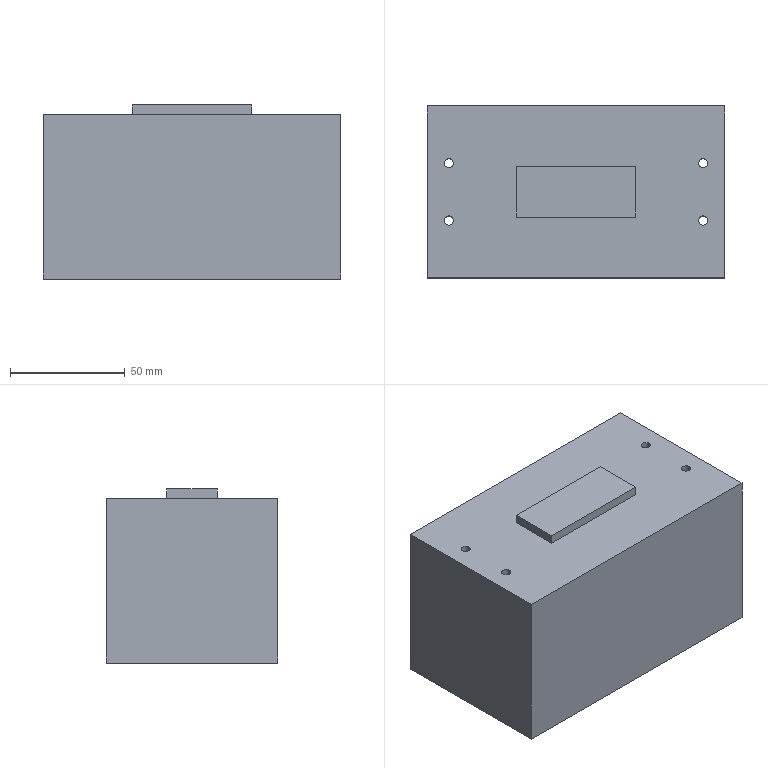Component | SolidWorks | Switch-1 | 1 solid | 19 faces | box 130 x 75 x 76 mm | volume 702957 mm3 | plane 11 | cylinder 8 | commonest cylinder face diameters 4 x8
build123d program:
from build123d import *

# Parameters (mm, degrees)
SKETCH1_W                 = 130
SKETCH1_H                 = 75
BOSS_EXTRUDE1_DEPTH       = 72
SKETCH2_W                 = 52
SKETCH2_H                 = 22
BOSS_EXTRUDE2_DEPTH       = 4
SKETCH3_R                 = 2
CUT_EXTRUDE1_DEPTH        = 80
LPATTERN1_COUNT           = 2
LPATTERN1_PITCH           = 25
LPATTERN2_COUNT           = 2
LPATTERN2_PITCH           = 111
LPATTERN2_COPY_1_SKETCH_R = 2
LPATTERN2_COPY_1_DEPTH    = 80


with BuildPart() as part:
    # Sketch1 → Boss-Extrude1 (new body)
    with BuildSketch(Plane.XY):
        Rectangle(SKETCH1_W, SKETCH1_H)
    extrude(amount=BOSS_EXTRUDE1_DEPTH)

    # Sketch2 → Boss-Extrude2 (add)
    with BuildSketch(Plane.XY.offset(72)):
        Rectangle(SKETCH2_W, SKETCH2_H)
    extrude(amount=BOSS_EXTRUDE2_DEPTH)

    # Sketch3 → Cut-Extrude1 (cut)
    with BuildSketch(Plane(origin=(0, 0, 0), x_dir=(-1, 0, 0), z_dir=(0, 0, -1))):
        with Locations((-55.5, -12.5)):
            Circle(SKETCH3_R)
    cut_extrude1 = extrude(amount=-CUT_EXTRUDE1_DEPTH, mode=Mode.SUBTRACT)

    # LPattern1: Cut-Extrude1 ×2
    with Locations(*[(0, i * LPATTERN1_PITCH, 0) for i in range(1, LPATTERN1_COUNT)]):
        add(cut_extrude1, mode=Mode.SUBTRACT)

    # LPattern2: Cut-Extrude1 ×2
    with Locations(*[(-i * LPATTERN2_PITCH, 0, 0) for i in range(1, LPATTERN2_COUNT)]):
        add(cut_extrude1, mode=Mode.SUBTRACT)

    # LPattern2 copy 1 sketch → LPattern2 copy 1 (cut)
    with BuildSketch(Plane(origin=(-111, 25, 0), x_dir=(-1, 0, 0), z_dir=(0, 0, -1))):
        with Locations((-55.5, -12.5)):
            Circle(LPATTERN2_COPY_1_SKETCH_R)
    extrude(amount=-LPATTERN2_COPY_1_DEPTH, mode=Mode.SUBTRACT)


solid = part.part

# Placed as in the assembly
solid = solid.moved(Location((172.727, 924.814, -141.5), (0, 0, 0)))
STEP:
#1=COLOUR_RGB('',0.7922,0.8196,0.9333);
#2=FILL_AREA_STYLE_COLOUR('',#1);
#3=FILL_AREA_STYLE('',(#2));
#4=SURFACE_STYLE_FILL_AREA(#3);
#5=SURFACE_SIDE_STYLE('',(#4));
#6=SURFACE_STYLE_USAGE(.BOTH.,#5);
#7=PRESENTATION_STYLE_ASSIGNMENT((#6));
#8=CARTESIAN_POINT('',(4.536,36.902,-2.736));
#9=VERTEX_POINT('',#8);
#10=CARTESIAN_POINT('',(4.694,36.902,-2.736));
#11=VERTEX_POINT('',#10);
#12=CARTESIAN_POINT('',(4.615,36.902,-2.736));
#13=DIRECTION('',(0.,0.,1.));
#14=DIRECTION('',(1.,0.,0.));
#15=AXIS2_PLACEMENT_3D('',#12,#13,#14);
#16=CIRCLE('',#15,0.07874);
#17=EDGE_CURVE('',#9,#11,#16,.T.);
#18=ORIENTED_EDGE('',*,*,#17,.T.);
#19=CARTESIAN_POINT('',(4.694,36.902,-5.571));
#20=VERTEX_POINT('',#19);
#21=CARTESIAN_POINT('',(4.694,36.902,-2.421));
#22=DIRECTION('',(0.,0.,-1.));
#23=VECTOR('',#22,39.37);
#24=LINE('',#21,#23);
#25=EDGE_CURVE('',#11,#20,#24,.T.);
#26=ORIENTED_EDGE('',*,*,#25,.T.);
#27=CARTESIAN_POINT('',(4.536,36.902,-5.571));
#28=VERTEX_POINT('',#27);
#29=CARTESIAN_POINT('',(4.615,36.902,-5.571));
#30=DIRECTION('',(0.,0.,-1.));
#31=DIRECTION('',(-1.,0.,0.));
#32=AXIS2_PLACEMENT_3D('',#29,#30,#31);
#33=CIRCLE('',#32,0.07874);
#34=EDGE_CURVE('',#20,#28,#33,.T.);
#35=ORIENTED_EDGE('',*,*,#34,.T.);
#36=CARTESIAN_POINT('',(4.536,36.902,-2.421));
#37=DIRECTION('',(0.,0.,-1.));
#38=VECTOR('',#37,39.37);
#39=LINE('',#36,#38);
#40=EDGE_CURVE('',#9,#28,#39,.T.);
#41=ORIENTED_EDGE('',*,*,#40,.F.);
#42=EDGE_LOOP('',(#18,#26,#35,#41));
#43=FACE_OUTER_BOUND('',#42,.T.);
#44=CARTESIAN_POINT('',(4.615,36.902,-2.421));
#45=DIRECTION('',(0.,0.,-1.));
#46=DIRECTION('',(-1.,0.,0.));
#47=AXIS2_PLACEMENT_3D('',#44,#45,#46);
#48=CYLINDRICAL_SURFACE('',#47,0.07874);
#49=ADVANCED_FACE('',(#43),#48,.F.);
#50=CARTESIAN_POINT('',(4.536,35.918,-2.736));
#51=VERTEX_POINT('',#50);
#52=CARTESIAN_POINT('',(4.694,35.918,-2.736));
#53=VERTEX_POINT('',#52);
#54=CARTESIAN_POINT('',(4.615,35.918,-2.736));
#55=DIRECTION('',(0.,0.,1.));
#56=DIRECTION('',(1.,0.,0.));
#57=AXIS2_PLACEMENT_3D('',#54,#55,#56);
#58=CIRCLE('',#57,0.07874);
#59=EDGE_CURVE('',#51,#53,#58,.T.);
#60=ORIENTED_EDGE('',*,*,#59,.T.);
#61=CARTESIAN_POINT('',(4.694,35.918,-5.571));
#62=VERTEX_POINT('',#61);
#63=CARTESIAN_POINT('',(4.694,35.918,-2.421));
#64=DIRECTION('',(0.,0.,-1.));
#65=VECTOR('',#64,39.37);
#66=LINE('',#63,#65);
#67=EDGE_CURVE('',#53,#62,#66,.T.);
#68=ORIENTED_EDGE('',*,*,#67,.T.);
#69=CARTESIAN_POINT('',(4.536,35.918,-5.571));
#70=VERTEX_POINT('',#69);
#71=CARTESIAN_POINT('',(4.615,35.918,-5.571));
#72=DIRECTION('',(0.,0.,-1.));
#73=DIRECTION('',(-1.,0.,0.));
#74=AXIS2_PLACEMENT_3D('',#71,#72,#73);
#75=CIRCLE('',#74,0.07874);
#76=EDGE_CURVE('',#62,#70,#75,.T.);
#77=ORIENTED_EDGE('',*,*,#76,.T.);
#78=CARTESIAN_POINT('',(4.536,35.918,-2.421));
#79=DIRECTION('',(0.,0.,-1.));
#80=VECTOR('',#79,39.37);
#81=LINE('',#78,#80);
#82=EDGE_CURVE('',#51,#70,#81,.T.);
#83=ORIENTED_EDGE('',*,*,#82,.F.);
#84=EDGE_LOOP('',(#60,#68,#77,#83));
#85=FACE_OUTER_BOUND('',#84,.T.);
#86=CARTESIAN_POINT('',(4.615,35.918,-2.421));
#87=DIRECTION('',(0.,0.,-1.));
#88=DIRECTION('',(-1.,0.,0.));
#89=AXIS2_PLACEMENT_3D('',#86,#87,#88);
#90=CYLINDRICAL_SURFACE('',#89,0.07874);
#91=ADVANCED_FACE('',(#85),#90,.F.);
#92=CARTESIAN_POINT('',(8.907,36.902,-2.736));
#93=VERTEX_POINT('',#92);
#94=CARTESIAN_POINT('',(9.064,36.902,-2.736));
#95=VERTEX_POINT('',#94);
#96=CARTESIAN_POINT('',(8.985,36.902,-2.736));
#97=DIRECTION('',(0.,0.,1.));
#98=DIRECTION('',(1.,0.,0.));
#99=AXIS2_PLACEMENT_3D('',#96,#97,#98);
#100=CIRCLE('',#99,0.07874);
#101=EDGE_CURVE('',#93,#95,#100,.T.);
#102=ORIENTED_EDGE('',*,*,#101,.T.);
#103=CARTESIAN_POINT('',(9.064,36.902,-5.571));
#104=VERTEX_POINT('',#103);
#105=CARTESIAN_POINT('',(9.064,36.902,-2.421));
#106=DIRECTION('',(0.,0.,-1.));
#107=VECTOR('',#106,39.37);
#108=LINE('',#105,#107);
#109=EDGE_CURVE('',#95,#104,#108,.T.);
#110=ORIENTED_EDGE('',*,*,#109,.T.);
#111=CARTESIAN_POINT('',(8.907,36.902,-5.571));
#112=VERTEX_POINT('',#111);
#113=CARTESIAN_POINT('',(8.985,36.902,-5.571));
#114=DIRECTION('',(0.,0.,-1.));
#115=DIRECTION('',(-1.,0.,0.));
#116=AXIS2_PLACEMENT_3D('',#113,#114,#115);
#117=CIRCLE('',#116,0.07874);
#118=EDGE_CURVE('',#104,#112,#117,.T.);
#119=ORIENTED_EDGE('',*,*,#118,.T.);
#120=CARTESIAN_POINT('',(8.907,36.902,-2.421));
#121=DIRECTION('',(0.,0.,-1.));
#122=VECTOR('',#121,39.37);
#123=LINE('',#120,#122);
#124=EDGE_CURVE('',#93,#112,#123,.T.);
#125=ORIENTED_EDGE('',*,*,#124,.F.);
#126=EDGE_LOOP('',(#102,#110,#119,#125));
#127=FACE_OUTER_BOUND('',#126,.T.);
#128=CARTESIAN_POINT('',(8.985,36.902,-2.421));
#129=DIRECTION('',(0.,0.,-1.));
#130=DIRECTION('',(-1.,0.,0.));
#131=AXIS2_PLACEMENT_3D('',#128,#129,#130);
#132=CYLINDRICAL_SURFACE('',#131,0.07874);
#133=ADVANCED_FACE('',(#127),#132,.F.);
#134=CARTESIAN_POINT('',(8.907,35.918,-2.736));
#135=VERTEX_POINT('',#134);
#136=CARTESIAN_POINT('',(9.064,35.918,-2.736));
#137=VERTEX_POINT('',#136);
#138=CARTESIAN_POINT('',(8.985,35.918,-2.736));
#139=DIRECTION('',(0.,0.,1.));
#140=DIRECTION('',(1.,0.,0.));
#141=AXIS2_PLACEMENT_3D('',#138,#139,#140);
#142=CIRCLE('',#141,0.07874);
#143=EDGE_CURVE('',#135,#137,#142,.T.);
#144=ORIENTED_EDGE('',*,*,#143,.T.);
#145=CARTESIAN_POINT('',(9.064,35.918,-5.571));
#146=VERTEX_POINT('',#145);
#147=CARTESIAN_POINT('',(9.064,35.918,-2.421));
#148=DIRECTION('',(0.,0.,-1.));
#149=VECTOR('',#148,39.37);
#150=LINE('',#147,#149);
#151=EDGE_CURVE('',#137,#146,#150,.T.);
#152=ORIENTED_EDGE('',*,*,#151,.T.);
#153=CARTESIAN_POINT('',(8.907,35.918,-5.571));
#154=VERTEX_POINT('',#153);
#155=CARTESIAN_POINT('',(8.985,35.918,-5.571));
#156=DIRECTION('',(0.,0.,-1.));
#157=DIRECTION('',(-1.,0.,0.));
#158=AXIS2_PLACEMENT_3D('',#155,#156,#157);
#159=CIRCLE('',#158,0.07874);
#160=EDGE_CURVE('',#146,#154,#159,.T.);
#161=ORIENTED_EDGE('',*,*,#160,.T.);
#162=CARTESIAN_POINT('',(8.907,35.918,-2.421));
#163=DIRECTION('',(0.,0.,-1.));
#164=VECTOR('',#163,39.37);
#165=LINE('',#162,#164);
#166=EDGE_CURVE('',#135,#154,#165,.T.);
#167=ORIENTED_EDGE('',*,*,#166,.F.);
#168=EDGE_LOOP('',(#144,#152,#161,#167));
#169=FACE_OUTER_BOUND('',#168,.T.);
#170=CARTESIAN_POINT('',(8.985,35.918,-2.421));
#171=DIRECTION('',(0.,0.,-1.));
#172=DIRECTION('',(-1.,0.,0.));
#173=AXIS2_PLACEMENT_3D('',#170,#171,#172);
#174=CYLINDRICAL_SURFACE('',#173,0.07874);
#175=ADVANCED_FACE('',(#169),#174,.F.);
#176=ORIENTED_EDGE('',*,*,#17,.F.);
#177=CARTESIAN_POINT('',(4.615,36.902,-2.736));
#178=DIRECTION('',(0.,0.,1.));
#179=DIRECTION('',(1.,0.,0.));
#180=AXIS2_PLACEMENT_3D('',#177,#178,#179);
#181=CIRCLE('',#180,0.07874);
#182=EDGE_CURVE('',#11,#9,#181,.T.);
#183=ORIENTED_EDGE('',*,*,#182,.F.);
#184=EDGE_LOOP('',(#176,#183));
#185=FACE_BOUND('',#184,.T.);
#186=ORIENTED_EDGE('',*,*,#59,.F.);
#187=CARTESIAN_POINT('',(4.615,35.918,-2.736));
#188=DIRECTION('',(0.,0.,1.));
#189=DIRECTION('',(1.,0.,0.));
#190=AXIS2_PLACEMENT_3D('',#187,#188,#189);
#191=CIRCLE('',#190,0.07874);
#192=EDGE_CURVE('',#53,#51,#191,.T.);
#193=ORIENTED_EDGE('',*,*,#192,.F.);
#194=EDGE_LOOP('',(#186,#193));
#195=FACE_BOUND('',#194,.T.);
#196=ORIENTED_EDGE('',*,*,#101,.F.);
#197=CARTESIAN_POINT('',(8.985,36.902,-2.736));
#198=DIRECTION('',(0.,0.,1.));
#199=DIRECTION('',(1.,0.,0.));
#200=AXIS2_PLACEMENT_3D('',#197,#198,#199);
#201=CIRCLE('',#200,0.07874);
#202=EDGE_CURVE('',#95,#93,#201,.T.);
#203=ORIENTED_EDGE('',*,*,#202,.F.);
#204=EDGE_LOOP('',(#196,#203));
#205=FACE_BOUND('',#204,.T.);
#206=ORIENTED_EDGE('',*,*,#143,.F.);
#207=CARTESIAN_POINT('',(8.985,35.918,-2.736));
#208=DIRECTION('',(0.,0.,1.));
#209=DIRECTION('',(1.,0.,0.));
#210=AXIS2_PLACEMENT_3D('',#207,#208,#209);
#211=CIRCLE('',#210,0.07874);
#212=EDGE_CURVE('',#137,#135,#211,.T.);
#213=ORIENTED_EDGE('',*,*,#212,.F.);
#214=EDGE_LOOP('',(#206,#213));
#215=FACE_BOUND('',#214,.T.);
#216=CARTESIAN_POINT('',(9.359,34.934,-2.736));
#217=VERTEX_POINT('',#216);
#218=CARTESIAN_POINT('',(9.359,37.886,-2.736));
#219=VERTEX_POINT('',#218);
#220=CARTESIAN_POINT('',(9.359,37.886,-2.736));
#221=DIRECTION('',(-0.,1.,0.));
#222=VECTOR('',#221,39.37);
#223=LINE('',#220,#222);
#224=EDGE_CURVE('',#217,#219,#223,.T.);
#225=ORIENTED_EDGE('',*,*,#224,.T.);
#226=CARTESIAN_POINT('',(4.241,37.886,-2.736));
#227=VERTEX_POINT('',#226);
#228=CARTESIAN_POINT('',(4.241,37.886,-2.736));
#229=DIRECTION('',(-1.,0.,0.));
#230=VECTOR('',#229,39.37);
#231=LINE('',#228,#230);
#232=EDGE_CURVE('',#219,#227,#231,.T.);
#233=ORIENTED_EDGE('',*,*,#232,.T.);
#234=CARTESIAN_POINT('',(4.241,34.934,-2.736));
#235=VERTEX_POINT('',#234);
#236=CARTESIAN_POINT('',(4.241,37.886,-2.736));
#237=DIRECTION('',(0.,-1.,0.));
#238=VECTOR('',#237,39.37);
#239=LINE('',#236,#238);
#240=EDGE_CURVE('',#227,#235,#239,.T.);
#241=ORIENTED_EDGE('',*,*,#240,.T.);
#242=CARTESIAN_POINT('',(4.241,34.934,-2.736));
#243=DIRECTION('',(1.,0.,0.));
#244=VECTOR('',#243,39.37);
#245=LINE('',#242,#244);
#246=EDGE_CURVE('',#235,#217,#245,.T.);
#247=ORIENTED_EDGE('',*,*,#246,.T.);
#248=EDGE_LOOP('',(#225,#233,#241,#247));
#249=FACE_OUTER_BOUND('',#248,.T.);
#250=CARTESIAN_POINT('',(7.824,36.843,-2.736));
#251=VERTEX_POINT('',#250);
#252=CARTESIAN_POINT('',(5.777,36.843,-2.736));
#253=VERTEX_POINT('',#252);
#254=CARTESIAN_POINT('',(5.777,36.843,-2.736));
#255=DIRECTION('',(-1.,0.,0.));
#256=VECTOR('',#255,39.37);
#257=LINE('',#254,#256);
#258=EDGE_CURVE('',#251,#253,#257,.T.);
#259=ORIENTED_EDGE('',*,*,#258,.F.);
#260=CARTESIAN_POINT('',(7.824,35.977,-2.736));
#261=VERTEX_POINT('',#260);
#262=CARTESIAN_POINT('',(7.824,36.843,-2.736));
#263=DIRECTION('',(0.,1.,0.));
#264=VECTOR('',#263,39.37);
#265=LINE('',#262,#264);
#266=EDGE_CURVE('',#261,#251,#265,.T.);
#267=ORIENTED_EDGE('',*,*,#266,.F.);
#268=CARTESIAN_POINT('',(5.777,35.977,-2.736));
#269=VERTEX_POINT('',#268);
#270=CARTESIAN_POINT('',(5.777,35.977,-2.736));
#271=DIRECTION('',(1.,0.,0.));
#272=VECTOR('',#271,39.37);
#273=LINE('',#270,#272);
#274=EDGE_CURVE('',#269,#261,#273,.T.);
#275=ORIENTED_EDGE('',*,*,#274,.F.);
#276=CARTESIAN_POINT('',(5.777,36.843,-2.736));
#277=DIRECTION('',(0.,-1.,0.));
#278=VECTOR('',#277,39.37);
#279=LINE('',#276,#278);
#280=EDGE_CURVE('',#253,#269,#279,.T.);
#281=ORIENTED_EDGE('',*,*,#280,.F.);
#282=EDGE_LOOP('',(#259,#267,#275,#281));
#283=FACE_BOUND('',#282,.T.);
#284=CARTESIAN_POINT('',(6.8,36.41,-2.736));
#285=DIRECTION('',(0.,0.,1.));
#286=DIRECTION('',(1.,0.,0.));
#287=AXIS2_PLACEMENT_3D('',#284,#285,#286);
#288=PLANE('',#287);
#289=ADVANCED_FACE('',(#185,#195,#205,#215,#249,#283),#288,.T.);
#290=CARTESIAN_POINT('',(9.359,34.934,-5.571));
#291=VERTEX_POINT('',#290);
#292=CARTESIAN_POINT('',(9.359,37.886,-5.571));
#293=VERTEX_POINT('',#292);
#294=CARTESIAN_POINT('',(9.359,37.886,-5.571));
#295=DIRECTION('',(-0.,1.,0.));
#296=VECTOR('',#295,39.37);
#297=LINE('',#294,#296);
#298=EDGE_CURVE('',#291,#293,#297,.T.);
#299=ORIENTED_EDGE('',*,*,#298,.T.);
#300=CARTESIAN_POINT('',(9.359,37.886,-2.736));
#301=DIRECTION('',(0.,0.,-1.));
#302=VECTOR('',#301,39.37);
#303=LINE('',#300,#302);
#304=EDGE_CURVE('',#219,#293,#303,.T.);
#305=ORIENTED_EDGE('',*,*,#304,.F.);
#306=ORIENTED_EDGE('',*,*,#224,.F.);
#307=CARTESIAN_POINT('',(9.359,34.934,-2.736));
#308=DIRECTION('',(0.,0.,-1.));
#309=VECTOR('',#308,39.37);
#310=LINE('',#307,#309);
#311=EDGE_CURVE('',#217,#291,#310,.T.);
#312=ORIENTED_EDGE('',*,*,#311,.T.);
#313=EDGE_LOOP('',(#299,#305,#306,#312));
#314=FACE_OUTER_BOUND('',#313,.T.);
#315=CARTESIAN_POINT('',(9.359,37.886,-2.736));
#316=DIRECTION('',(-1.,-0.,0.));
#317=DIRECTION('',(0.,-1.,0.));
#318=AXIS2_PLACEMENT_3D('',#315,#316,#317);
#319=PLANE('',#318);
#320=ADVANCED_FACE('',(#314),#319,.F.);
#321=CARTESIAN_POINT('',(4.241,37.886,-5.571));
#322=VERTEX_POINT('',#321);
#323=CARTESIAN_POINT('',(4.241,37.886,-5.571));
#324=DIRECTION('',(-1.,0.,0.));
#325=VECTOR('',#324,39.37);
#326=LINE('',#323,#325);
#327=EDGE_CURVE('',#293,#322,#326,.T.);
#328=ORIENTED_EDGE('',*,*,#327,.T.);
#329=CARTESIAN_POINT('',(4.241,37.886,-2.736));
#330=DIRECTION('',(0.,0.,-1.));
#331=VECTOR('',#330,39.37);
#332=LINE('',#329,#331);
#333=EDGE_CURVE('',#227,#322,#332,.T.);
#334=ORIENTED_EDGE('',*,*,#333,.F.);
#335=ORIENTED_EDGE('',*,*,#232,.F.);
#336=ORIENTED_EDGE('',*,*,#304,.T.);
#337=EDGE_LOOP('',(#328,#334,#335,#336));
#338=FACE_OUTER_BOUND('',#337,.T.);
#339=CARTESIAN_POINT('',(4.241,37.886,-2.736));
#340=DIRECTION('',(0.,-1.,0.));
#341=DIRECTION('',(0.,0.,-1.));
#342=AXIS2_PLACEMENT_3D('',#339,#340,#341);
#343=PLANE('',#342);
#344=ADVANCED_FACE('',(#338),#343,.F.);
#345=CARTESIAN_POINT('',(4.241,34.934,-5.571));
#346=VERTEX_POINT('',#345);
#347=CARTESIAN_POINT('',(4.241,37.886,-5.571));
#348=DIRECTION('',(0.,-1.,0.));
#349=VECTOR('',#348,39.37);
#350=LINE('',#347,#349);
#351=EDGE_CURVE('',#322,#346,#350,.T.);
#352=ORIENTED_EDGE('',*,*,#351,.T.);
#353=CARTESIAN_POINT('',(4.241,34.934,-2.736));
#354=DIRECTION('',(0.,0.,-1.));
#355=VECTOR('',#354,39.37);
#356=LINE('',#353,#355);
#357=EDGE_CURVE('',#235,#346,#356,.T.);
#358=ORIENTED_EDGE('',*,*,#357,.F.);
#359=ORIENTED_EDGE('',*,*,#240,.F.);
#360=ORIENTED_EDGE('',*,*,#333,.T.);
#361=EDGE_LOOP('',(#352,#358,#359,#360));
#362=FACE_OUTER_BOUND('',#361,.T.);
#363=CARTESIAN_POINT('',(4.241,37.886,-2.736));
#364=DIRECTION('',(1.,0.,0.));
#365=DIRECTION('',(-0.,1.,0.));
#366=AXIS2_PLACEMENT_3D('',#363,#364,#365);
#367=PLANE('',#366);
#368=ADVANCED_FACE('',(#362),#367,.F.);
#369=CARTESIAN_POINT('',(4.241,34.934,-5.571));
#370=DIRECTION('',(1.,0.,0.));
#371=VECTOR('',#370,39.37);
#372=LINE('',#369,#371);
#373=EDGE_CURVE('',#346,#291,#372,.T.);
#374=ORIENTED_EDGE('',*,*,#373,.T.);
#375=ORIENTED_EDGE('',*,*,#311,.F.);
#376=ORIENTED_EDGE('',*,*,#246,.F.);
#377=ORIENTED_EDGE('',*,*,#357,.T.);
#378=EDGE_LOOP('',(#374,#375,#376,#377));
#379=FACE_OUTER_BOUND('',#378,.T.);
#380=CARTESIAN_POINT('',(4.241,34.934,-2.736));
#381=DIRECTION('',(0.,1.,0.));
#382=DIRECTION('',(0.,0.,1.));
#383=AXIS2_PLACEMENT_3D('',#380,#381,#382);
#384=PLANE('',#383);
#385=ADVANCED_FACE('',(#379),#384,.F.);
#386=CARTESIAN_POINT('',(4.615,36.902,-5.571));
#387=DIRECTION('',(0.,0.,-1.));
#388=DIRECTION('',(-1.,0.,0.));
#389=AXIS2_PLACEMENT_3D('',#386,#387,#388);
#390=CIRCLE('',#389,0.07874);
#391=EDGE_CURVE('',#28,#20,#390,.T.);
#392=ORIENTED_EDGE('',*,*,#391,.F.);
#393=ORIENTED_EDGE('',*,*,#34,.F.);
#394=EDGE_LOOP('',(#392,#393));
#395=FACE_BOUND('',#394,.T.);
#396=CARTESIAN_POINT('',(4.615,35.918,-5.571));
#397=DIRECTION('',(0.,0.,-1.));
#398=DIRECTION('',(-1.,0.,0.));
#399=AXIS2_PLACEMENT_3D('',#396,#397,#398);
#400=CIRCLE('',#399,0.07874);
#401=EDGE_CURVE('',#70,#62,#400,.T.);
#402=ORIENTED_EDGE('',*,*,#401,.F.);
#403=ORIENTED_EDGE('',*,*,#76,.F.);
#404=EDGE_LOOP('',(#402,#403));
#405=FACE_BOUND('',#404,.T.);
#406=CARTESIAN_POINT('',(8.985,36.902,-5.571));
#407=DIRECTION('',(0.,0.,-1.));
#408=DIRECTION('',(-1.,0.,0.));
#409=AXIS2_PLACEMENT_3D('',#406,#407,#408);
#410=CIRCLE('',#409,0.07874);
#411=EDGE_CURVE('',#112,#104,#410,.T.);
#412=ORIENTED_EDGE('',*,*,#411,.F.);
#413=ORIENTED_EDGE('',*,*,#118,.F.);
#414=EDGE_LOOP('',(#412,#413));
#415=FACE_BOUND('',#414,.T.);
#416=CARTESIAN_POINT('',(8.985,35.918,-5.571));
#417=DIRECTION('',(0.,0.,-1.));
#418=DIRECTION('',(-1.,0.,0.));
#419=AXIS2_PLACEMENT_3D('',#416,#417,#418);
#420=CIRCLE('',#419,0.07874);
#421=EDGE_CURVE('',#154,#146,#420,.T.);
#422=ORIENTED_EDGE('',*,*,#421,.F.);
#423=ORIENTED_EDGE('',*,*,#160,.F.);
#424=EDGE_LOOP('',(#422,#423));
#425=FACE_BOUND('',#424,.T.);
#426=ORIENTED_EDGE('',*,*,#298,.F.);
#427=ORIENTED_EDGE('',*,*,#373,.F.);
#428=ORIENTED_EDGE('',*,*,#351,.F.);
#429=ORIENTED_EDGE('',*,*,#327,.F.);
#430=EDGE_LOOP('',(#426,#427,#428,#429));
#431=FACE_OUTER_BOUND('',#430,.T.);
#432=CARTESIAN_POINT('',(6.8,36.41,-5.571));
#433=DIRECTION('',(0.,0.,1.));
#434=DIRECTION('',(1.,0.,0.));
#435=AXIS2_PLACEMENT_3D('',#432,#433,#434);
#436=PLANE('',#435);
#437=ADVANCED_FACE('',(#395,#405,#415,#425,#431),#436,.F.);
#438=ORIENTED_EDGE('',*,*,#266,.T.);
#439=CARTESIAN_POINT('',(7.824,36.843,-2.579));
#440=VERTEX_POINT('',#439);
#441=CARTESIAN_POINT('',(7.824,36.843,-2.579));
#442=DIRECTION('',(0.,0.,-1.));
#443=VECTOR('',#442,39.37);
#444=LINE('',#441,#443);
#445=EDGE_CURVE('',#440,#251,#444,.T.);
#446=ORIENTED_EDGE('',*,*,#445,.F.);
#447=CARTESIAN_POINT('',(7.824,35.977,-2.579));
#448=VERTEX_POINT('',#447);
#449=CARTESIAN_POINT('',(7.824,36.843,-2.579));
#450=DIRECTION('',(0.,1.,0.));
#451=VECTOR('',#450,39.37);
#452=LINE('',#449,#451);
#453=EDGE_CURVE('',#448,#440,#452,.T.);
#454=ORIENTED_EDGE('',*,*,#453,.F.);
#455=CARTESIAN_POINT('',(7.824,35.977,-2.579));
#456=DIRECTION('',(0.,0.,-1.));
#457=VECTOR('',#456,39.37);
#458=LINE('',#455,#457);
#459=EDGE_CURVE('',#448,#261,#458,.T.);
#460=ORIENTED_EDGE('',*,*,#459,.T.);
#461=EDGE_LOOP('',(#438,#446,#454,#460));
#462=FACE_OUTER_BOUND('',#461,.T.);
#463=CARTESIAN_POINT('',(7.824,36.843,-2.579));
#464=DIRECTION('',(-1.,0.,0.));
#465=DIRECTION('',(-0.,-1.,0.));
#466=AXIS2_PLACEMENT_3D('',#463,#464,#465);
#467=PLANE('',#466);
#468=ADVANCED_FACE('',(#462),#467,.F.);
#469=ORIENTED_EDGE('',*,*,#258,.T.);
#470=CARTESIAN_POINT('',(5.777,36.843,-2.579));
#471=VERTEX_POINT('',#470);
#472=CARTESIAN_POINT('',(5.777,36.843,-2.579));
#473=DIRECTION('',(0.,0.,-1.));
#474=VECTOR('',#473,39.37);
#475=LINE('',#472,#474);
#476=EDGE_CURVE('',#471,#253,#475,.T.);
#477=ORIENTED_EDGE('',*,*,#476,.F.);
#478=CARTESIAN_POINT('',(5.777,36.843,-2.579));
#479=DIRECTION('',(-1.,0.,0.));
#480=VECTOR('',#479,39.37);
#481=LINE('',#478,#480);
#482=EDGE_CURVE('',#440,#471,#481,.T.);
#483=ORIENTED_EDGE('',*,*,#482,.F.);
#484=ORIENTED_EDGE('',*,*,#445,.T.);
#485=EDGE_LOOP('',(#469,#477,#483,#484));
#486=FACE_OUTER_BOUND('',#485,.T.);
#487=CARTESIAN_POINT('',(5.777,36.843,-2.579));
#488=DIRECTION('',(0.,-1.,0.));
#489=DIRECTION('',(0.,0.,-1.));
#490=AXIS2_PLACEMENT_3D('',#487,#488,#489);
#491=PLANE('',#490);
#492=ADVANCED_FACE('',(#486),#491,.F.);
#493=ORIENTED_EDGE('',*,*,#280,.T.);
#494=CARTESIAN_POINT('',(5.777,35.977,-2.579));
#495=VERTEX_POINT('',#494);
#496=CARTESIAN_POINT('',(5.777,35.977,-2.579));
#497=DIRECTION('',(0.,0.,-1.));
#498=VECTOR('',#497,39.37);
#499=LINE('',#496,#498);
#500=EDGE_CURVE('',#495,#269,#499,.T.);
#501=ORIENTED_EDGE('',*,*,#500,.F.);
#502=CARTESIAN_POINT('',(5.777,36.843,-2.579));
#503=DIRECTION('',(0.,-1.,0.));
#504=VECTOR('',#503,39.37);
#505=LINE('',#502,#504);
#506=EDGE_CURVE('',#471,#495,#505,.T.);
#507=ORIENTED_EDGE('',*,*,#506,.F.);
#508=ORIENTED_EDGE('',*,*,#476,.T.);
#509=EDGE_LOOP('',(#493,#501,#507,#508));
#510=FACE_OUTER_BOUND('',#509,.T.);
#511=CARTESIAN_POINT('',(5.777,36.843,-2.579));
#512=DIRECTION('',(1.,0.,0.));
#513=DIRECTION('',(-0.,1.,0.));
#514=AXIS2_PLACEMENT_3D('',#511,#512,#513);
#515=PLANE('',#514);
#516=ADVANCED_FACE('',(#510),#515,.F.);
#517=ORIENTED_EDGE('',*,*,#274,.T.);
#518=ORIENTED_EDGE('',*,*,#459,.F.);
#519=CARTESIAN_POINT('',(5.777,35.977,-2.579));
#520=DIRECTION('',(1.,0.,0.));
#521=VECTOR('',#520,39.37);
#522=LINE('',#519,#521);
#523=EDGE_CURVE('',#495,#448,#522,.T.);
#524=ORIENTED_EDGE('',*,*,#523,.F.);
#525=ORIENTED_EDGE('',*,*,#500,.T.);
#526=EDGE_LOOP('',(#517,#518,#524,#525));
#527=FACE_OUTER_BOUND('',#526,.T.);
#528=CARTESIAN_POINT('',(5.777,35.977,-2.579));
#529=DIRECTION('',(0.,1.,0.));
#530=DIRECTION('',(0.,0.,1.));
#531=AXIS2_PLACEMENT_3D('',#528,#529,#530);
#532=PLANE('',#531);
#533=ADVANCED_FACE('',(#527),#532,.F.);
#534=ORIENTED_EDGE('',*,*,#453,.T.);
#535=ORIENTED_EDGE('',*,*,#482,.T.);
#536=ORIENTED_EDGE('',*,*,#506,.T.);
#537=ORIENTED_EDGE('',*,*,#523,.T.);
#538=EDGE_LOOP('',(#534,#535,#536,#537));
#539=FACE_OUTER_BOUND('',#538,.T.);
#540=CARTESIAN_POINT('',(6.8,36.41,-2.579));
#541=DIRECTION('',(0.,0.,1.));
#542=DIRECTION('',(1.,0.,0.));
#543=AXIS2_PLACEMENT_3D('',#540,#541,#542);
#544=PLANE('',#543);
#545=ADVANCED_FACE('',(#539),#544,.T.);
#546=ORIENTED_EDGE('',*,*,#151,.F.);
#547=ORIENTED_EDGE('',*,*,#212,.T.);
#548=ORIENTED_EDGE('',*,*,#166,.T.);
#549=ORIENTED_EDGE('',*,*,#421,.T.);
#550=EDGE_LOOP('',(#546,#547,#548,#549));
#551=FACE_OUTER_BOUND('',#550,.T.);
#552=CARTESIAN_POINT('',(8.985,35.918,-2.421));
#553=DIRECTION('',(0.,0.,-1.));
#554=DIRECTION('',(-1.,0.,0.));
#555=AXIS2_PLACEMENT_3D('',#552,#553,#554);
#556=CYLINDRICAL_SURFACE('',#555,0.07874);
#557=ADVANCED_FACE('',(#551),#556,.F.);
#558=ORIENTED_EDGE('',*,*,#109,.F.);
#559=ORIENTED_EDGE('',*,*,#202,.T.);
#560=ORIENTED_EDGE('',*,*,#124,.T.);
#561=ORIENTED_EDGE('',*,*,#411,.T.);
#562=EDGE_LOOP('',(#558,#559,#560,#561));
#563=FACE_OUTER_BOUND('',#562,.T.);
#564=CARTESIAN_POINT('',(8.985,36.902,-2.421));
#565=DIRECTION('',(0.,0.,-1.));
#566=DIRECTION('',(-1.,0.,0.));
#567=AXIS2_PLACEMENT_3D('',#564,#565,#566);
#568=CYLINDRICAL_SURFACE('',#567,0.07874);
#569=ADVANCED_FACE('',(#563),#568,.F.);
#570=ORIENTED_EDGE('',*,*,#67,.F.);
#571=ORIENTED_EDGE('',*,*,#192,.T.);
#572=ORIENTED_EDGE('',*,*,#82,.T.);
#573=ORIENTED_EDGE('',*,*,#401,.T.);
#574=EDGE_LOOP('',(#570,#571,#572,#573));
#575=FACE_OUTER_BOUND('',#574,.T.);
#576=CARTESIAN_POINT('',(4.615,35.918,-2.421));
#577=DIRECTION('',(0.,0.,-1.));
#578=DIRECTION('',(-1.,0.,0.));
#579=AXIS2_PLACEMENT_3D('',#576,#577,#578);
#580=CYLINDRICAL_SURFACE('',#579,0.07874);
#581=ADVANCED_FACE('',(#575),#580,.F.);
#582=ORIENTED_EDGE('',*,*,#25,.F.);
#583=ORIENTED_EDGE('',*,*,#182,.T.);
#584=ORIENTED_EDGE('',*,*,#40,.T.);
#585=ORIENTED_EDGE('',*,*,#391,.T.);
#586=EDGE_LOOP('',(#582,#583,#584,#585));
#587=FACE_OUTER_BOUND('',#586,.T.);
#588=CARTESIAN_POINT('',(4.615,36.902,-2.421));
#589=DIRECTION('',(0.,0.,-1.));
#590=DIRECTION('',(-1.,0.,0.));
#591=AXIS2_PLACEMENT_3D('',#588,#589,#590);
#592=CYLINDRICAL_SURFACE('',#591,0.07874);
#593=ADVANCED_FACE('',(#587),#592,.F.);
#594=CLOSED_SHELL('',(#49,#91,#133,#175,#289,#320,#344,#368,#385,#437,#468,#492,#516,#533,#545,#557,#569,#581,#593));
#595=MANIFOLD_SOLID_BREP('',#594);
#596=STYLED_ITEM('',(#7),#595);
#597=PRESENTATION_LAYER_ASSIGNMENT('','',(#596));
#598=CARTESIAN_POINT('',(0.,0.,0.));
#599=DIRECTION('',(0.,0.,1.));
#600=DIRECTION('',(1.,0.,0.));
#601=AXIS2_PLACEMENT_3D('',#598,#599,#600);
#602=(LENGTH_UNIT()NAMED_UNIT(*)SI_UNIT($,.METRE.));
#603=LENGTH_MEASURE_WITH_UNIT(LENGTH_MEASURE(0.0254),#602);
#604=DIMENSIONAL_EXPONENTS(1.,0.,0.,0.,0.,0.,0.);
#605=(CONVERSION_BASED_UNIT('',#603)LENGTH_UNIT()NAMED_UNIT(#604));
#606=UNCERTAINTY_MEASURE_WITH_UNIT(LENGTH_MEASURE(0.00001),#605,'','');
#607=(NAMED_UNIT(*)PLANE_ANGLE_UNIT()SI_UNIT($,.RADIAN.));
#608=(NAMED_UNIT(*)SI_UNIT($,.STERADIAN.)SOLID_ANGLE_UNIT());
#609=(GEOMETRIC_REPRESENTATION_CONTEXT(3)GLOBAL_UNCERTAINTY_ASSIGNED_CONTEXT((#606))GLOBAL_UNIT_ASSIGNED_CONTEXT((#605,#607,#608))REPRESENTATION_CONTEXT('',''));
#610=ADVANCED_BREP_SHAPE_REPRESENTATION('',(#595,#601),#609);
#611=(LENGTH_UNIT()NAMED_UNIT(*)SI_UNIT($,.METRE.));
#612=LENGTH_MEASURE_WITH_UNIT(LENGTH_MEASURE(0.0254),#611);
#613=DIMENSIONAL_EXPONENTS(1.,0.,0.,0.,0.,0.,0.);
#614=(CONVERSION_BASED_UNIT('',#612)LENGTH_UNIT()NAMED_UNIT(#613));
#615=UNCERTAINTY_MEASURE_WITH_UNIT(LENGTH_MEASURE(0.00001),#614,'','');
#616=(NAMED_UNIT(*)PLANE_ANGLE_UNIT()SI_UNIT($,.RADIAN.));
#617=(NAMED_UNIT(*)SI_UNIT($,.STERADIAN.)SOLID_ANGLE_UNIT());
#618=(GEOMETRIC_REPRESENTATION_CONTEXT(3)GLOBAL_UNCERTAINTY_ASSIGNED_CONTEXT((#615))GLOBAL_UNIT_ASSIGNED_CONTEXT((#614,#616,#617))REPRESENTATION_CONTEXT('',''));
#619=MECHANICAL_DESIGN_GEOMETRIC_PRESENTATION_REPRESENTATION('',(#596),#618);